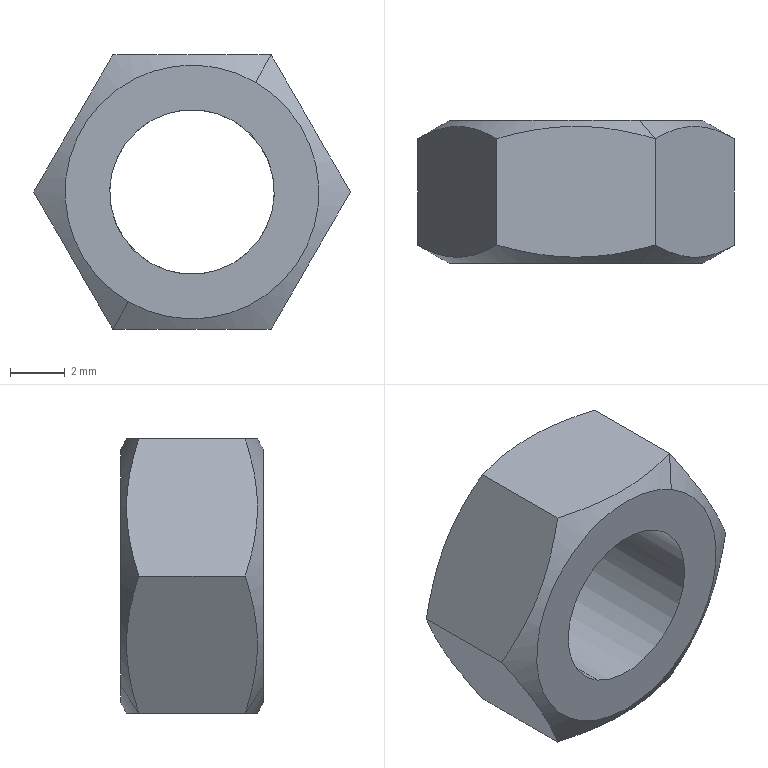Component | SolidWorks | ClampingAssembly-1_M6-N-1 | 1 solid | 14 faces | box 11.55 x 5.2 x 10 mm | volume 295 mm3 | plane 8 | cone 4 | cylinder 2 | commonest cylinder face diameters 6 x2 | material Standard Part
STEP:
#1=CARTESIAN_POINT('',(-0.2776,4.616,-1.728));
#2=VERTEX_POINT('',#1);
#3=CARTESIAN_POINT('',(-0.3957,4.616,-1.933));
#4=VERTEX_POINT('',#3);
#5=CARTESIAN_POINT('',(-0.3366,4.616,-1.831));
#6=DIRECTION('',(0.,-1.,0.));
#7=DIRECTION('',(-0.5,0.,-0.866));
#8=AXIS2_PLACEMENT_3D('',#5,#6,#7);
#9=CIRCLE('',#8,0.1181);
#10=EDGE_CURVE('',#2,#4,#9,.T.);
#11=ORIENTED_EDGE('',*,*,#10,.F.);
#12=CARTESIAN_POINT('',(-0.2776,4.411,-1.728));
#13=VERTEX_POINT('',#12);
#14=CARTESIAN_POINT('',(-0.2776,4.616,-1.728));
#15=DIRECTION('',(0.,-1.,0.));
#16=VECTOR('',#15,39.37);
#17=LINE('',#14,#16);
#18=EDGE_CURVE('',#2,#13,#17,.T.);
#19=ORIENTED_EDGE('',*,*,#18,.T.);
#20=CARTESIAN_POINT('',(-0.3957,4.411,-1.933));
#21=VERTEX_POINT('',#20);
#22=CARTESIAN_POINT('',(-0.2776,4.411,-1.728));
#23=CARTESIAN_POINT('',(-0.291,4.411,-1.721));
#24=CARTESIAN_POINT('',(-0.3059,4.411,-1.716));
#25=CARTESIAN_POINT('',(-0.3366,4.411,-1.712));
#26=CARTESIAN_POINT('',(-0.3523,4.411,-1.713));
#27=CARTESIAN_POINT('',(-0.3821,4.411,-1.721));
#28=CARTESIAN_POINT('',(-0.3963,4.411,-1.728));
#29=CARTESIAN_POINT('',(-0.4208,4.411,-1.746));
#30=CARTESIAN_POINT('',(-0.4312,4.411,-1.758));
#31=CARTESIAN_POINT('',(-0.4467,4.411,-1.785));
#32=CARTESIAN_POINT('',(-0.4517,4.411,-1.8));
#33=CARTESIAN_POINT('',(-0.4558,4.411,-1.831));
#34=CARTESIAN_POINT('',(-0.4547,4.411,-1.846));
#35=CARTESIAN_POINT('',(-0.4467,4.411,-1.876));
#36=CARTESIAN_POINT('',(-0.4398,4.411,-1.89));
#37=CARTESIAN_POINT('',(-0.4209,4.411,-1.915));
#38=CARTESIAN_POINT('',(-0.4091,4.411,-1.925));
#39=CARTESIAN_POINT('',(-0.3957,4.411,-1.933));
#40=B_SPLINE_CURVE_WITH_KNOTS('',3,(#22,#23,#24,#25,#26,#27,#28,#29,#30,#31,#32,#33,#34,#35,#36,#37,#38,#39),.UNSPECIFIED.,.F.,.F.,(4,2,2,2,2,2,2,2,4),(0.5,0.5625,0.625,0.6875,0.75,0.8125,0.875,0.9375,1.),.UNSPECIFIED.);
#41=EDGE_CURVE('',#13,#21,#40,.T.);
#42=ORIENTED_EDGE('',*,*,#41,.T.);
#43=CARTESIAN_POINT('',(-0.3957,4.616,-1.933));
#44=DIRECTION('',(0.,-1.,0.));
#45=VECTOR('',#44,39.37);
#46=LINE('',#43,#45);
#47=EDGE_CURVE('',#4,#21,#46,.T.);
#48=ORIENTED_EDGE('',*,*,#47,.F.);
#49=EDGE_LOOP('',(#11,#19,#42,#48));
#50=FACE_OUTER_BOUND('',#49,.T.);
#51=CARTESIAN_POINT('',(-0.3366,4.616,-1.831));
#52=DIRECTION('',(0.,-1.,0.));
#53=DIRECTION('',(-0.5,0.,-0.866));
#54=AXIS2_PLACEMENT_3D('',#51,#52,#53);
#55=CYLINDRICAL_SURFACE('',#54,0.1181);
#56=ADVANCED_FACE('',(#50),#55,.F.);
#57=CARTESIAN_POINT('',(-0.2456,4.616,-1.673));
#58=VERTEX_POINT('',#57);
#59=CARTESIAN_POINT('',(-0.4277,4.616,-1.988));
#60=VERTEX_POINT('',#59);
#61=CARTESIAN_POINT('',(-0.3366,4.616,-1.831));
#62=DIRECTION('',(-0.,1.,-0.));
#63=DIRECTION('',(-0.5,0.,-0.866));
#64=AXIS2_PLACEMENT_3D('',#61,#62,#63);
#65=CIRCLE('',#64,0.1821);
#66=EDGE_CURVE('',#58,#60,#65,.T.);
#67=ORIENTED_EDGE('',*,*,#66,.F.);
#68=CARTESIAN_POINT('',(-0.223,4.589,-1.634));
#69=VERTEX_POINT('',#68);
#70=CARTESIAN_POINT('',(-0.2229,4.589,-1.634));
#71=DIRECTION('',(0.433,-0.5,0.75));
#72=VECTOR('',#71,39.37);
#73=LINE('',#70,#72);
#74=EDGE_CURVE('',#58,#69,#73,.T.);
#75=ORIENTED_EDGE('',*,*,#74,.T.);
#76=CARTESIAN_POINT('',(-0.1093,4.589,-1.831));
#77=VERTEX_POINT('',#76);
#78=CARTESIAN_POINT('',(-0.223,4.589,-1.634));
#79=CARTESIAN_POINT('',(-0.2044,4.6,-1.666));
#80=CARTESIAN_POINT('',(-0.1856,4.607,-1.699));
#81=CARTESIAN_POINT('',(-0.1614,4.607,-1.74));
#82=CARTESIAN_POINT('',(-0.1566,4.607,-1.749));
#83=CARTESIAN_POINT('',(-0.147,4.605,-1.766));
#84=CARTESIAN_POINT('',(-0.1422,4.604,-1.774));
#85=CARTESIAN_POINT('',(-0.128,4.599,-1.798));
#86=CARTESIAN_POINT('',(-0.1186,4.595,-1.815));
#87=CARTESIAN_POINT('',(-0.1093,4.589,-1.831));
#88=B_SPLINE_CURVE_WITH_KNOTS('',3,(#78,#79,#80,#81,#82,#83,#84,#85,#86,#87),.UNSPECIFIED.,.F.,.F.,(4,2,2,2,4),(0.,0.002915,0.003644,0.004373,0.005831),.UNSPECIFIED.);
#89=EDGE_CURVE('',#69,#77,#88,.T.);
#90=ORIENTED_EDGE('',*,*,#89,.T.);
#91=CARTESIAN_POINT('',(-0.223,4.589,-2.028));
#92=VERTEX_POINT('',#91);
#93=CARTESIAN_POINT('',(-0.1093,4.589,-1.831));
#94=CARTESIAN_POINT('',(-0.1279,4.6,-1.863));
#95=CARTESIAN_POINT('',(-0.1467,4.607,-1.895));
#96=CARTESIAN_POINT('',(-0.1709,4.607,-1.937));
#97=CARTESIAN_POINT('',(-0.1757,4.607,-1.946));
#98=CARTESIAN_POINT('',(-0.1853,4.605,-1.962));
#99=CARTESIAN_POINT('',(-0.1901,4.604,-1.971));
#100=CARTESIAN_POINT('',(-0.2043,4.599,-1.995));
#101=CARTESIAN_POINT('',(-0.2137,4.595,-2.011));
#102=CARTESIAN_POINT('',(-0.223,4.589,-2.028));
#103=B_SPLINE_CURVE_WITH_KNOTS('',3,(#93,#94,#95,#96,#97,#98,#99,#100,#101,#102),.UNSPECIFIED.,.F.,.F.,(4,2,2,2,4),(0.,0.002915,0.003644,0.004373,0.005831),.UNSPECIFIED.);
#104=EDGE_CURVE('',#77,#92,#103,.T.);
#105=ORIENTED_EDGE('',*,*,#104,.T.);
#106=CARTESIAN_POINT('',(-0.4503,4.589,-2.028));
#107=VERTEX_POINT('',#106);
#108=CARTESIAN_POINT('',(-0.223,4.589,-2.028));
#109=CARTESIAN_POINT('',(-0.2601,4.6,-2.028));
#110=CARTESIAN_POINT('',(-0.2978,4.607,-2.028));
#111=CARTESIAN_POINT('',(-0.3461,4.607,-2.028));
#112=CARTESIAN_POINT('',(-0.3558,4.607,-2.028));
#113=CARTESIAN_POINT('',(-0.375,4.605,-2.028));
#114=CARTESIAN_POINT('',(-0.3845,4.604,-2.028));
#115=CARTESIAN_POINT('',(-0.413,4.599,-2.028));
#116=CARTESIAN_POINT('',(-0.4317,4.595,-2.028));
#117=CARTESIAN_POINT('',(-0.4503,4.589,-2.028));
#118=B_SPLINE_CURVE_WITH_KNOTS('',3,(#108,#109,#110,#111,#112,#113,#114,#115,#116,#117),.UNSPECIFIED.,.F.,.F.,(4,2,2,2,4),(0.,0.002915,0.003644,0.004373,0.005831),.UNSPECIFIED.);
#119=EDGE_CURVE('',#92,#107,#118,.T.);
#120=ORIENTED_EDGE('',*,*,#119,.T.);
#121=CARTESIAN_POINT('',(-0.4504,4.589,-2.028));
#122=DIRECTION('',(-0.433,-0.5,-0.75));
#123=VECTOR('',#122,39.37);
#124=LINE('',#121,#123);
#125=EDGE_CURVE('',#60,#107,#124,.T.);
#126=ORIENTED_EDGE('',*,*,#125,.F.);
#127=EDGE_LOOP('',(#67,#75,#90,#105,#120,#126));
#128=FACE_OUTER_BOUND('',#127,.T.);
#129=CARTESIAN_POINT('',(-0.3366,4.589,-1.831));
#130=DIRECTION('',(0.,-1.,0.));
#131=DIRECTION('',(-0.5,0.,-0.866));
#132=AXIS2_PLACEMENT_3D('',#129,#130,#131);
#133=CONICAL_SURFACE('',#132,0.2276,1.047);
#134=ADVANCED_FACE('',(#128),#133,.T.);
#135=CARTESIAN_POINT('',(-0.2456,4.411,-1.673));
#136=VERTEX_POINT('',#135);
#137=CARTESIAN_POINT('',(-0.4277,4.411,-1.988));
#138=VERTEX_POINT('',#137);
#139=CARTESIAN_POINT('',(-0.3366,4.411,-1.831));
#140=DIRECTION('',(-0.,1.,-0.));
#141=DIRECTION('',(0.5,0.,0.866));
#142=AXIS2_PLACEMENT_3D('',#139,#140,#141);
#143=CIRCLE('',#142,0.1821);
#144=EDGE_CURVE('',#136,#138,#143,.T.);
#145=ORIENTED_EDGE('',*,*,#144,.T.);
#146=CARTESIAN_POINT('',(-0.4503,4.437,-2.028));
#147=VERTEX_POINT('',#146);
#148=CARTESIAN_POINT('',(-0.4504,4.437,-2.028));
#149=DIRECTION('',(-0.433,0.5,-0.75));
#150=VECTOR('',#149,39.37);
#151=LINE('',#148,#150);
#152=EDGE_CURVE('',#138,#147,#151,.T.);
#153=ORIENTED_EDGE('',*,*,#152,.T.);
#154=CARTESIAN_POINT('',(-0.223,4.437,-2.028));
#155=VERTEX_POINT('',#154);
#156=CARTESIAN_POINT('',(-0.223,4.437,-2.028));
#157=CARTESIAN_POINT('',(-0.2601,4.426,-2.028));
#158=CARTESIAN_POINT('',(-0.2978,4.419,-2.028));
#159=CARTESIAN_POINT('',(-0.3461,4.419,-2.028));
#160=CARTESIAN_POINT('',(-0.3558,4.42,-2.028));
#161=CARTESIAN_POINT('',(-0.375,4.421,-2.028));
#162=CARTESIAN_POINT('',(-0.3845,4.423,-2.028));
#163=CARTESIAN_POINT('',(-0.413,4.427,-2.028));
#164=CARTESIAN_POINT('',(-0.4317,4.432,-2.028));
#165=CARTESIAN_POINT('',(-0.4503,4.437,-2.028));
#166=B_SPLINE_CURVE_WITH_KNOTS('',3,(#156,#157,#158,#159,#160,#161,#162,#163,#164,#165),.UNSPECIFIED.,.F.,.F.,(4,2,2,2,4),(0.,0.002915,0.003644,0.004373,0.005831),.UNSPECIFIED.);
#167=EDGE_CURVE('',#155,#147,#166,.T.);
#168=ORIENTED_EDGE('',*,*,#167,.F.);
#169=CARTESIAN_POINT('',(-0.1093,4.437,-1.831));
#170=VERTEX_POINT('',#169);
#171=CARTESIAN_POINT('',(-0.1093,4.437,-1.831));
#172=CARTESIAN_POINT('',(-0.1279,4.426,-1.863));
#173=CARTESIAN_POINT('',(-0.1467,4.419,-1.895));
#174=CARTESIAN_POINT('',(-0.1709,4.419,-1.937));
#175=CARTESIAN_POINT('',(-0.1757,4.42,-1.946));
#176=CARTESIAN_POINT('',(-0.1853,4.421,-1.962));
#177=CARTESIAN_POINT('',(-0.1901,4.423,-1.971));
#178=CARTESIAN_POINT('',(-0.2043,4.427,-1.995));
#179=CARTESIAN_POINT('',(-0.2137,4.432,-2.011));
#180=CARTESIAN_POINT('',(-0.223,4.437,-2.028));
#181=B_SPLINE_CURVE_WITH_KNOTS('',3,(#171,#172,#173,#174,#175,#176,#177,#178,#179,#180),.UNSPECIFIED.,.F.,.F.,(4,2,2,2,4),(0.,0.002915,0.003644,0.004373,0.005831),.UNSPECIFIED.);
#182=EDGE_CURVE('',#170,#155,#181,.T.);
#183=ORIENTED_EDGE('',*,*,#182,.F.);
#184=CARTESIAN_POINT('',(-0.223,4.437,-1.634));
#185=VERTEX_POINT('',#184);
#186=CARTESIAN_POINT('',(-0.223,4.437,-1.634));
#187=CARTESIAN_POINT('',(-0.2044,4.426,-1.666));
#188=CARTESIAN_POINT('',(-0.1856,4.419,-1.699));
#189=CARTESIAN_POINT('',(-0.1614,4.419,-1.74));
#190=CARTESIAN_POINT('',(-0.1566,4.42,-1.749));
#191=CARTESIAN_POINT('',(-0.147,4.421,-1.766));
#192=CARTESIAN_POINT('',(-0.1422,4.423,-1.774));
#193=CARTESIAN_POINT('',(-0.128,4.427,-1.798));
#194=CARTESIAN_POINT('',(-0.1186,4.432,-1.815));
#195=CARTESIAN_POINT('',(-0.1093,4.437,-1.831));
#196=B_SPLINE_CURVE_WITH_KNOTS('',3,(#186,#187,#188,#189,#190,#191,#192,#193,#194,#195),.UNSPECIFIED.,.F.,.F.,(4,2,2,2,4),(0.,0.002915,0.003644,0.004373,0.005831),.UNSPECIFIED.);
#197=EDGE_CURVE('',#185,#170,#196,.T.);
#198=ORIENTED_EDGE('',*,*,#197,.F.);
#199=CARTESIAN_POINT('',(-0.2229,4.437,-1.634));
#200=DIRECTION('',(0.433,0.5,0.75));
#201=VECTOR('',#200,39.37);
#202=LINE('',#199,#201);
#203=EDGE_CURVE('',#136,#185,#202,.T.);
#204=ORIENTED_EDGE('',*,*,#203,.F.);
#205=EDGE_LOOP('',(#145,#153,#168,#183,#198,#204));
#206=FACE_OUTER_BOUND('',#205,.T.);
#207=CARTESIAN_POINT('',(-0.3366,4.437,-1.831));
#208=DIRECTION('',(-0.,1.,-0.));
#209=DIRECTION('',(0.5,0.,0.866));
#210=AXIS2_PLACEMENT_3D('',#207,#208,#209);
#211=CONICAL_SURFACE('',#210,0.2276,1.047);
#212=ADVANCED_FACE('',(#206),#211,.T.);
#213=CARTESIAN_POINT('',(-0.3366,4.616,-1.831));
#214=DIRECTION('',(0.,-1.,0.));
#215=DIRECTION('',(-0.5,0.,-0.866));
#216=AXIS2_PLACEMENT_3D('',#213,#214,#215);
#217=CIRCLE('',#216,0.1181);
#218=EDGE_CURVE('',#4,#2,#217,.T.);
#219=ORIENTED_EDGE('',*,*,#218,.T.);
#220=ORIENTED_EDGE('',*,*,#10,.T.);
#221=EDGE_LOOP('',(#219,#220));
#222=FACE_BOUND('',#221,.T.);
#223=CARTESIAN_POINT('',(-0.3366,4.616,-1.831));
#224=DIRECTION('',(-0.,1.,-0.));
#225=DIRECTION('',(-0.5,0.,-0.866));
#226=AXIS2_PLACEMENT_3D('',#223,#224,#225);
#227=CIRCLE('',#226,0.1821);
#228=EDGE_CURVE('',#60,#58,#227,.T.);
#229=ORIENTED_EDGE('',*,*,#228,.T.);
#230=ORIENTED_EDGE('',*,*,#66,.T.);
#231=EDGE_LOOP('',(#229,#230));
#232=FACE_OUTER_BOUND('',#231,.T.);
#233=CARTESIAN_POINT('',(-0.6776,4.616,-1.634));
#234=DIRECTION('',(-0.,1.,-0.));
#235=DIRECTION('',(0.5,0.,0.866));
#236=AXIS2_PLACEMENT_3D('',#233,#234,#235);
#237=PLANE('',#236);
#238=ADVANCED_FACE('',(#222,#232),#237,.T.);
#239=ORIENTED_EDGE('',*,*,#74,.F.);
#240=ORIENTED_EDGE('',*,*,#228,.F.);
#241=ORIENTED_EDGE('',*,*,#125,.T.);
#242=CARTESIAN_POINT('',(-0.5639,4.589,-1.831));
#243=VERTEX_POINT('',#242);
#244=CARTESIAN_POINT('',(-0.4503,4.589,-2.028));
#245=CARTESIAN_POINT('',(-0.4689,4.6,-1.995));
#246=CARTESIAN_POINT('',(-0.4877,4.607,-1.963));
#247=CARTESIAN_POINT('',(-0.5118,4.607,-1.921));
#248=CARTESIAN_POINT('',(-0.5167,4.607,-1.913));
#249=CARTESIAN_POINT('',(-0.5263,4.605,-1.896));
#250=CARTESIAN_POINT('',(-0.5311,4.604,-1.888));
#251=CARTESIAN_POINT('',(-0.5453,4.599,-1.863));
#252=CARTESIAN_POINT('',(-0.5547,4.595,-1.847));
#253=CARTESIAN_POINT('',(-0.5639,4.589,-1.831));
#254=B_SPLINE_CURVE_WITH_KNOTS('',3,(#244,#245,#246,#247,#248,#249,#250,#251,#252,#253),.UNSPECIFIED.,.F.,.F.,(4,2,2,2,4),(0.,0.002915,0.003644,0.004373,0.005831),.UNSPECIFIED.);
#255=EDGE_CURVE('',#107,#243,#254,.T.);
#256=ORIENTED_EDGE('',*,*,#255,.T.);
#257=CARTESIAN_POINT('',(-0.4503,4.589,-1.634));
#258=VERTEX_POINT('',#257);
#259=CARTESIAN_POINT('',(-0.5639,4.589,-1.831));
#260=CARTESIAN_POINT('',(-0.5454,4.6,-1.799));
#261=CARTESIAN_POINT('',(-0.5266,4.607,-1.766));
#262=CARTESIAN_POINT('',(-0.5024,4.607,-1.724));
#263=CARTESIAN_POINT('',(-0.4975,4.607,-1.716));
#264=CARTESIAN_POINT('',(-0.4879,4.605,-1.699));
#265=CARTESIAN_POINT('',(-0.4832,4.604,-1.691));
#266=CARTESIAN_POINT('',(-0.469,4.599,-1.666));
#267=CARTESIAN_POINT('',(-0.4596,4.595,-1.65));
#268=CARTESIAN_POINT('',(-0.4503,4.589,-1.634));
#269=B_SPLINE_CURVE_WITH_KNOTS('',3,(#259,#260,#261,#262,#263,#264,#265,#266,#267,#268),.UNSPECIFIED.,.F.,.F.,(4,2,2,2,4),(0.,0.002915,0.003644,0.004373,0.005831),.UNSPECIFIED.);
#270=EDGE_CURVE('',#243,#258,#269,.T.);
#271=ORIENTED_EDGE('',*,*,#270,.T.);
#272=CARTESIAN_POINT('',(-0.4503,4.589,-1.634));
#273=CARTESIAN_POINT('',(-0.4132,4.6,-1.634));
#274=CARTESIAN_POINT('',(-0.3755,4.607,-1.634));
#275=CARTESIAN_POINT('',(-0.3272,4.607,-1.634));
#276=CARTESIAN_POINT('',(-0.3175,4.607,-1.634));
#277=CARTESIAN_POINT('',(-0.2983,4.605,-1.634));
#278=CARTESIAN_POINT('',(-0.2888,4.604,-1.634));
#279=CARTESIAN_POINT('',(-0.2603,4.599,-1.634));
#280=CARTESIAN_POINT('',(-0.2416,4.595,-1.634));
#281=CARTESIAN_POINT('',(-0.223,4.589,-1.634));
#282=B_SPLINE_CURVE_WITH_KNOTS('',3,(#272,#273,#274,#275,#276,#277,#278,#279,#280,#281),.UNSPECIFIED.,.F.,.F.,(4,2,2,2,4),(0.,0.002915,0.003644,0.004373,0.005831),.UNSPECIFIED.);
#283=EDGE_CURVE('',#258,#69,#282,.T.);
#284=ORIENTED_EDGE('',*,*,#283,.T.);
#285=EDGE_LOOP('',(#239,#240,#241,#256,#271,#284));
#286=FACE_OUTER_BOUND('',#285,.T.);
#287=CARTESIAN_POINT('',(-0.3366,4.589,-1.831));
#288=DIRECTION('',(0.,-1.,0.));
#289=DIRECTION('',(-0.5,0.,-0.866));
#290=AXIS2_PLACEMENT_3D('',#287,#288,#289);
#291=CONICAL_SURFACE('',#290,0.2276,1.047);
#292=ADVANCED_FACE('',(#286),#291,.T.);
#293=ORIENTED_EDGE('',*,*,#119,.F.);
#294=CARTESIAN_POINT('',(-0.223,4.616,-2.028));
#295=DIRECTION('',(0.,-1.,0.));
#296=VECTOR('',#295,39.37);
#297=LINE('',#294,#296);
#298=EDGE_CURVE('',#92,#155,#297,.T.);
#299=ORIENTED_EDGE('',*,*,#298,.T.);
#300=ORIENTED_EDGE('',*,*,#167,.T.);
#301=CARTESIAN_POINT('',(-0.4503,4.616,-2.028));
#302=DIRECTION('',(-0.,1.,-0.));
#303=VECTOR('',#302,39.37);
#304=LINE('',#301,#303);
#305=EDGE_CURVE('',#147,#107,#304,.T.);
#306=ORIENTED_EDGE('',*,*,#305,.T.);
#307=EDGE_LOOP('',(#293,#299,#300,#306));
#308=FACE_OUTER_BOUND('',#307,.T.);
#309=CARTESIAN_POINT('',(-0.4503,4.616,-2.028));
#310=DIRECTION('',(0.,-0.,-1.));
#311=DIRECTION('',(1.,0.,0.));
#312=AXIS2_PLACEMENT_3D('',#309,#310,#311);
#313=PLANE('',#312);
#314=ADVANCED_FACE('',(#308),#313,.T.);
#315=ORIENTED_EDGE('',*,*,#104,.F.);
#316=CARTESIAN_POINT('',(-0.1093,4.616,-1.831));
#317=DIRECTION('',(0.,-1.,0.));
#318=VECTOR('',#317,39.37);
#319=LINE('',#316,#318);
#320=EDGE_CURVE('',#77,#170,#319,.T.);
#321=ORIENTED_EDGE('',*,*,#320,.T.);
#322=ORIENTED_EDGE('',*,*,#182,.T.);
#323=ORIENTED_EDGE('',*,*,#298,.F.);
#324=EDGE_LOOP('',(#315,#321,#322,#323));
#325=FACE_OUTER_BOUND('',#324,.T.);
#326=CARTESIAN_POINT('',(-0.223,4.616,-2.028));
#327=DIRECTION('',(0.866,0.,-0.5));
#328=DIRECTION('',(0.,-1.,0.));
#329=AXIS2_PLACEMENT_3D('',#326,#327,#328);
#330=PLANE('',#329);
#331=ADVANCED_FACE('',(#325),#330,.T.);
#332=ORIENTED_EDGE('',*,*,#89,.F.);
#333=CARTESIAN_POINT('',(-0.223,4.616,-1.634));
#334=DIRECTION('',(0.,-1.,0.));
#335=VECTOR('',#334,39.37);
#336=LINE('',#333,#335);
#337=EDGE_CURVE('',#69,#185,#336,.T.);
#338=ORIENTED_EDGE('',*,*,#337,.T.);
#339=ORIENTED_EDGE('',*,*,#197,.T.);
#340=ORIENTED_EDGE('',*,*,#320,.F.);
#341=EDGE_LOOP('',(#332,#338,#339,#340));
#342=FACE_OUTER_BOUND('',#341,.T.);
#343=CARTESIAN_POINT('',(-0.1093,4.616,-1.831));
#344=DIRECTION('',(0.866,0.,0.5));
#345=DIRECTION('',(-0.5,0.,0.866));
#346=AXIS2_PLACEMENT_3D('',#343,#344,#345);
#347=PLANE('',#346);
#348=ADVANCED_FACE('',(#342),#347,.T.);
#349=ORIENTED_EDGE('',*,*,#283,.F.);
#350=CARTESIAN_POINT('',(-0.4503,4.437,-1.634));
#351=VERTEX_POINT('',#350);
#352=CARTESIAN_POINT('',(-0.4503,4.616,-1.634));
#353=DIRECTION('',(0.,-1.,0.));
#354=VECTOR('',#353,39.37);
#355=LINE('',#352,#354);
#356=EDGE_CURVE('',#258,#351,#355,.T.);
#357=ORIENTED_EDGE('',*,*,#356,.T.);
#358=CARTESIAN_POINT('',(-0.4503,4.437,-1.634));
#359=CARTESIAN_POINT('',(-0.4132,4.426,-1.634));
#360=CARTESIAN_POINT('',(-0.3755,4.419,-1.634));
#361=CARTESIAN_POINT('',(-0.3272,4.419,-1.634));
#362=CARTESIAN_POINT('',(-0.3175,4.42,-1.634));
#363=CARTESIAN_POINT('',(-0.2983,4.421,-1.634));
#364=CARTESIAN_POINT('',(-0.2888,4.423,-1.634));
#365=CARTESIAN_POINT('',(-0.2603,4.427,-1.634));
#366=CARTESIAN_POINT('',(-0.2416,4.432,-1.634));
#367=CARTESIAN_POINT('',(-0.223,4.437,-1.634));
#368=B_SPLINE_CURVE_WITH_KNOTS('',3,(#358,#359,#360,#361,#362,#363,#364,#365,#366,#367),.UNSPECIFIED.,.F.,.F.,(4,2,2,2,4),(0.,0.002915,0.003644,0.004373,0.005831),.UNSPECIFIED.);
#369=EDGE_CURVE('',#351,#185,#368,.T.);
#370=ORIENTED_EDGE('',*,*,#369,.T.);
#371=ORIENTED_EDGE('',*,*,#337,.F.);
#372=EDGE_LOOP('',(#349,#357,#370,#371));
#373=FACE_OUTER_BOUND('',#372,.T.);
#374=CARTESIAN_POINT('',(-0.223,4.616,-1.634));
#375=DIRECTION('',(-0.,0.,1.));
#376=DIRECTION('',(-1.,-0.,-0.));
#377=AXIS2_PLACEMENT_3D('',#374,#375,#376);
#378=PLANE('',#377);
#379=ADVANCED_FACE('',(#373),#378,.T.);
#380=ORIENTED_EDGE('',*,*,#270,.F.);
#381=CARTESIAN_POINT('',(-0.5639,4.437,-1.831));
#382=VERTEX_POINT('',#381);
#383=CARTESIAN_POINT('',(-0.5639,4.616,-1.831));
#384=DIRECTION('',(0.,-1.,0.));
#385=VECTOR('',#384,39.37);
#386=LINE('',#383,#385);
#387=EDGE_CURVE('',#243,#382,#386,.T.);
#388=ORIENTED_EDGE('',*,*,#387,.T.);
#389=CARTESIAN_POINT('',(-0.5639,4.437,-1.831));
#390=CARTESIAN_POINT('',(-0.5454,4.426,-1.799));
#391=CARTESIAN_POINT('',(-0.5266,4.419,-1.766));
#392=CARTESIAN_POINT('',(-0.5024,4.419,-1.724));
#393=CARTESIAN_POINT('',(-0.4975,4.42,-1.716));
#394=CARTESIAN_POINT('',(-0.4879,4.421,-1.699));
#395=CARTESIAN_POINT('',(-0.4832,4.423,-1.691));
#396=CARTESIAN_POINT('',(-0.469,4.427,-1.666));
#397=CARTESIAN_POINT('',(-0.4596,4.432,-1.65));
#398=CARTESIAN_POINT('',(-0.4503,4.437,-1.634));
#399=B_SPLINE_CURVE_WITH_KNOTS('',3,(#389,#390,#391,#392,#393,#394,#395,#396,#397,#398),.UNSPECIFIED.,.F.,.F.,(4,2,2,2,4),(0.,0.002915,0.003644,0.004373,0.005831),.UNSPECIFIED.);
#400=EDGE_CURVE('',#382,#351,#399,.T.);
#401=ORIENTED_EDGE('',*,*,#400,.T.);
#402=ORIENTED_EDGE('',*,*,#356,.F.);
#403=EDGE_LOOP('',(#380,#388,#401,#402));
#404=FACE_OUTER_BOUND('',#403,.T.);
#405=CARTESIAN_POINT('',(-0.4503,4.616,-1.634));
#406=DIRECTION('',(-0.866,-0.,0.5));
#407=DIRECTION('',(-0.5,-0.,-0.866));
#408=AXIS2_PLACEMENT_3D('',#405,#406,#407);
#409=PLANE('',#408);
#410=ADVANCED_FACE('',(#404),#409,.T.);
#411=ORIENTED_EDGE('',*,*,#255,.F.);
#412=ORIENTED_EDGE('',*,*,#305,.F.);
#413=CARTESIAN_POINT('',(-0.4503,4.437,-2.028));
#414=CARTESIAN_POINT('',(-0.4689,4.426,-1.995));
#415=CARTESIAN_POINT('',(-0.4877,4.419,-1.963));
#416=CARTESIAN_POINT('',(-0.5118,4.419,-1.921));
#417=CARTESIAN_POINT('',(-0.5167,4.42,-1.913));
#418=CARTESIAN_POINT('',(-0.5263,4.421,-1.896));
#419=CARTESIAN_POINT('',(-0.5311,4.423,-1.888));
#420=CARTESIAN_POINT('',(-0.5453,4.427,-1.863));
#421=CARTESIAN_POINT('',(-0.5547,4.432,-1.847));
#422=CARTESIAN_POINT('',(-0.5639,4.437,-1.831));
#423=B_SPLINE_CURVE_WITH_KNOTS('',3,(#413,#414,#415,#416,#417,#418,#419,#420,#421,#422),.UNSPECIFIED.,.F.,.F.,(4,2,2,2,4),(0.,0.002915,0.003644,0.004373,0.005831),.UNSPECIFIED.);
#424=EDGE_CURVE('',#147,#382,#423,.T.);
#425=ORIENTED_EDGE('',*,*,#424,.T.);
#426=ORIENTED_EDGE('',*,*,#387,.F.);
#427=EDGE_LOOP('',(#411,#412,#425,#426));
#428=FACE_OUTER_BOUND('',#427,.T.);
#429=CARTESIAN_POINT('',(-0.5639,4.616,-1.831));
#430=DIRECTION('',(-0.866,-0.,-0.5));
#431=DIRECTION('',(0.5,-0.,-0.866));
#432=AXIS2_PLACEMENT_3D('',#429,#430,#431);
#433=PLANE('',#432);
#434=ADVANCED_FACE('',(#428),#433,.T.);
#435=ORIENTED_EDGE('',*,*,#152,.F.);
#436=CARTESIAN_POINT('',(-0.3366,4.411,-1.831));
#437=DIRECTION('',(-0.,1.,-0.));
#438=DIRECTION('',(0.5,0.,0.866));
#439=AXIS2_PLACEMENT_3D('',#436,#437,#438);
#440=CIRCLE('',#439,0.1821);
#441=EDGE_CURVE('',#138,#136,#440,.T.);
#442=ORIENTED_EDGE('',*,*,#441,.T.);
#443=ORIENTED_EDGE('',*,*,#203,.T.);
#444=ORIENTED_EDGE('',*,*,#369,.F.);
#445=ORIENTED_EDGE('',*,*,#400,.F.);
#446=ORIENTED_EDGE('',*,*,#424,.F.);
#447=EDGE_LOOP('',(#435,#442,#443,#444,#445,#446));
#448=FACE_OUTER_BOUND('',#447,.T.);
#449=CARTESIAN_POINT('',(-0.3366,4.437,-1.831));
#450=DIRECTION('',(-0.,1.,-0.));
#451=DIRECTION('',(0.5,0.,0.866));
#452=AXIS2_PLACEMENT_3D('',#449,#450,#451);
#453=CONICAL_SURFACE('',#452,0.2276,1.047);
#454=ADVANCED_FACE('',(#448),#453,.T.);
#455=ORIENTED_EDGE('',*,*,#144,.F.);
#456=ORIENTED_EDGE('',*,*,#441,.F.);
#457=EDGE_LOOP('',(#455,#456));
#458=FACE_OUTER_BOUND('',#457,.T.);
#459=CARTESIAN_POINT('',(-0.3957,4.411,-1.933));
#460=CARTESIAN_POINT('',(-0.3823,4.411,-1.941));
#461=CARTESIAN_POINT('',(-0.3674,4.411,-1.946));
#462=CARTESIAN_POINT('',(-0.3367,4.411,-1.95));
#463=CARTESIAN_POINT('',(-0.321,4.411,-1.949));
#464=CARTESIAN_POINT('',(-0.2911,4.411,-1.941));
#465=CARTESIAN_POINT('',(-0.277,4.411,-1.934));
#466=CARTESIAN_POINT('',(-0.2525,4.411,-1.915));
#467=CARTESIAN_POINT('',(-0.2421,4.411,-1.903));
#468=CARTESIAN_POINT('',(-0.2266,4.411,-1.876));
#469=CARTESIAN_POINT('',(-0.2216,4.411,-1.861));
#470=CARTESIAN_POINT('',(-0.2175,4.411,-1.831));
#471=CARTESIAN_POINT('',(-0.2186,4.411,-1.815));
#472=CARTESIAN_POINT('',(-0.2266,4.411,-1.785));
#473=CARTESIAN_POINT('',(-0.2335,4.411,-1.771));
#474=CARTESIAN_POINT('',(-0.2524,4.411,-1.747));
#475=CARTESIAN_POINT('',(-0.2642,4.411,-1.736));
#476=CARTESIAN_POINT('',(-0.2776,4.411,-1.728));
#477=B_SPLINE_CURVE_WITH_KNOTS('',3,(#459,#460,#461,#462,#463,#464,#465,#466,#467,#468,#469,#470,#471,#472,#473,#474,#475,#476),.UNSPECIFIED.,.F.,.F.,(4,2,2,2,2,2,2,2,4),(0.,0.0625,0.125,0.1875,0.25,0.3125,0.375,0.4375,0.5),.UNSPECIFIED.);
#478=EDGE_CURVE('',#21,#13,#477,.T.);
#479=ORIENTED_EDGE('',*,*,#478,.F.);
#480=ORIENTED_EDGE('',*,*,#41,.F.);
#481=EDGE_LOOP('',(#479,#480));
#482=FACE_BOUND('',#481,.T.);
#483=CARTESIAN_POINT('',(-0.6776,4.411,-1.634));
#484=DIRECTION('',(-0.,1.,-0.));
#485=DIRECTION('',(0.5,0.,0.866));
#486=AXIS2_PLACEMENT_3D('',#483,#484,#485);
#487=PLANE('',#486);
#488=ADVANCED_FACE('',(#458,#482),#487,.F.);
#489=ORIENTED_EDGE('',*,*,#18,.F.);
#490=ORIENTED_EDGE('',*,*,#218,.F.);
#491=ORIENTED_EDGE('',*,*,#47,.T.);
#492=ORIENTED_EDGE('',*,*,#478,.T.);
#493=EDGE_LOOP('',(#489,#490,#491,#492));
#494=FACE_OUTER_BOUND('',#493,.T.);
#495=CARTESIAN_POINT('',(-0.3366,4.616,-1.831));
#496=DIRECTION('',(0.,-1.,0.));
#497=DIRECTION('',(-0.5,0.,-0.866));
#498=AXIS2_PLACEMENT_3D('',#495,#496,#497);
#499=CYLINDRICAL_SURFACE('',#498,0.1181);
#500=ADVANCED_FACE('',(#494),#499,.F.);
#501=CLOSED_SHELL('',(#56,#134,#212,#238,#292,#314,#331,#348,#379,#410,#434,#454,#488,#500));
#502=MANIFOLD_SOLID_BREP('',#501);
#503=CARTESIAN_POINT('',(0.,0.,0.));
#504=DIRECTION('',(0.,0.,1.));
#505=DIRECTION('',(1.,0.,0.));
#506=AXIS2_PLACEMENT_3D('',#503,#504,#505);
#507=(LENGTH_UNIT()NAMED_UNIT(*)SI_UNIT($,.METRE.));
#508=LENGTH_MEASURE_WITH_UNIT(LENGTH_MEASURE(0.0254),#507);
#509=DIMENSIONAL_EXPONENTS(1.,0.,0.,0.,0.,0.,0.);
#510=(CONVERSION_BASED_UNIT('',#508)LENGTH_UNIT()NAMED_UNIT(#509));
#511=UNCERTAINTY_MEASURE_WITH_UNIT(LENGTH_MEASURE(0.00001),#510,'','');
#512=(NAMED_UNIT(*)PLANE_ANGLE_UNIT()SI_UNIT($,.RADIAN.));
#513=(NAMED_UNIT(*)SI_UNIT($,.STERADIAN.)SOLID_ANGLE_UNIT());
#514=(GEOMETRIC_REPRESENTATION_CONTEXT(3)GLOBAL_UNCERTAINTY_ASSIGNED_CONTEXT((#511))GLOBAL_UNIT_ASSIGNED_CONTEXT((#510,#512,#513))REPRESENTATION_CONTEXT('',''));
#515=ADVANCED_BREP_SHAPE_REPRESENTATION('',(#502,#506),#514);
#516=COLOUR_RGB('',0.7922,0.8196,0.9333);
#517=FILL_AREA_STYLE_COLOUR('',#516);
#518=FILL_AREA_STYLE('',(#517));
#519=SURFACE_STYLE_FILL_AREA(#518);
#520=SURFACE_SIDE_STYLE('',(#519));
#521=SURFACE_STYLE_USAGE(.BOTH.,#520);
#522=PRESENTATION_STYLE_ASSIGNMENT((#521));
#523=STYLED_ITEM('',(#522),#502);
#524=(LENGTH_UNIT()NAMED_UNIT(*)SI_UNIT($,.METRE.));
#525=LENGTH_MEASURE_WITH_UNIT(LENGTH_MEASURE(0.0254),#524);
#526=DIMENSIONAL_EXPONENTS(1.,0.,0.,0.,0.,0.,0.);
#527=(CONVERSION_BASED_UNIT('',#525)LENGTH_UNIT()NAMED_UNIT(#526));
#528=UNCERTAINTY_MEASURE_WITH_UNIT(LENGTH_MEASURE(0.00001),#527,'','');
#529=(NAMED_UNIT(*)PLANE_ANGLE_UNIT()SI_UNIT($,.RADIAN.));
#530=(NAMED_UNIT(*)SI_UNIT($,.STERADIAN.)SOLID_ANGLE_UNIT());
#531=(GEOMETRIC_REPRESENTATION_CONTEXT(3)GLOBAL_UNCERTAINTY_ASSIGNED_CONTEXT((#528))GLOBAL_UNIT_ASSIGNED_CONTEXT((#527,#529,#530))REPRESENTATION_CONTEXT('',''));
#532=MECHANICAL_DESIGN_GEOMETRIC_PRESENTATION_REPRESENTATION('',(#523),#531);
#533=PRESENTATION_LAYER_ASSIGNMENT('','',(#523));